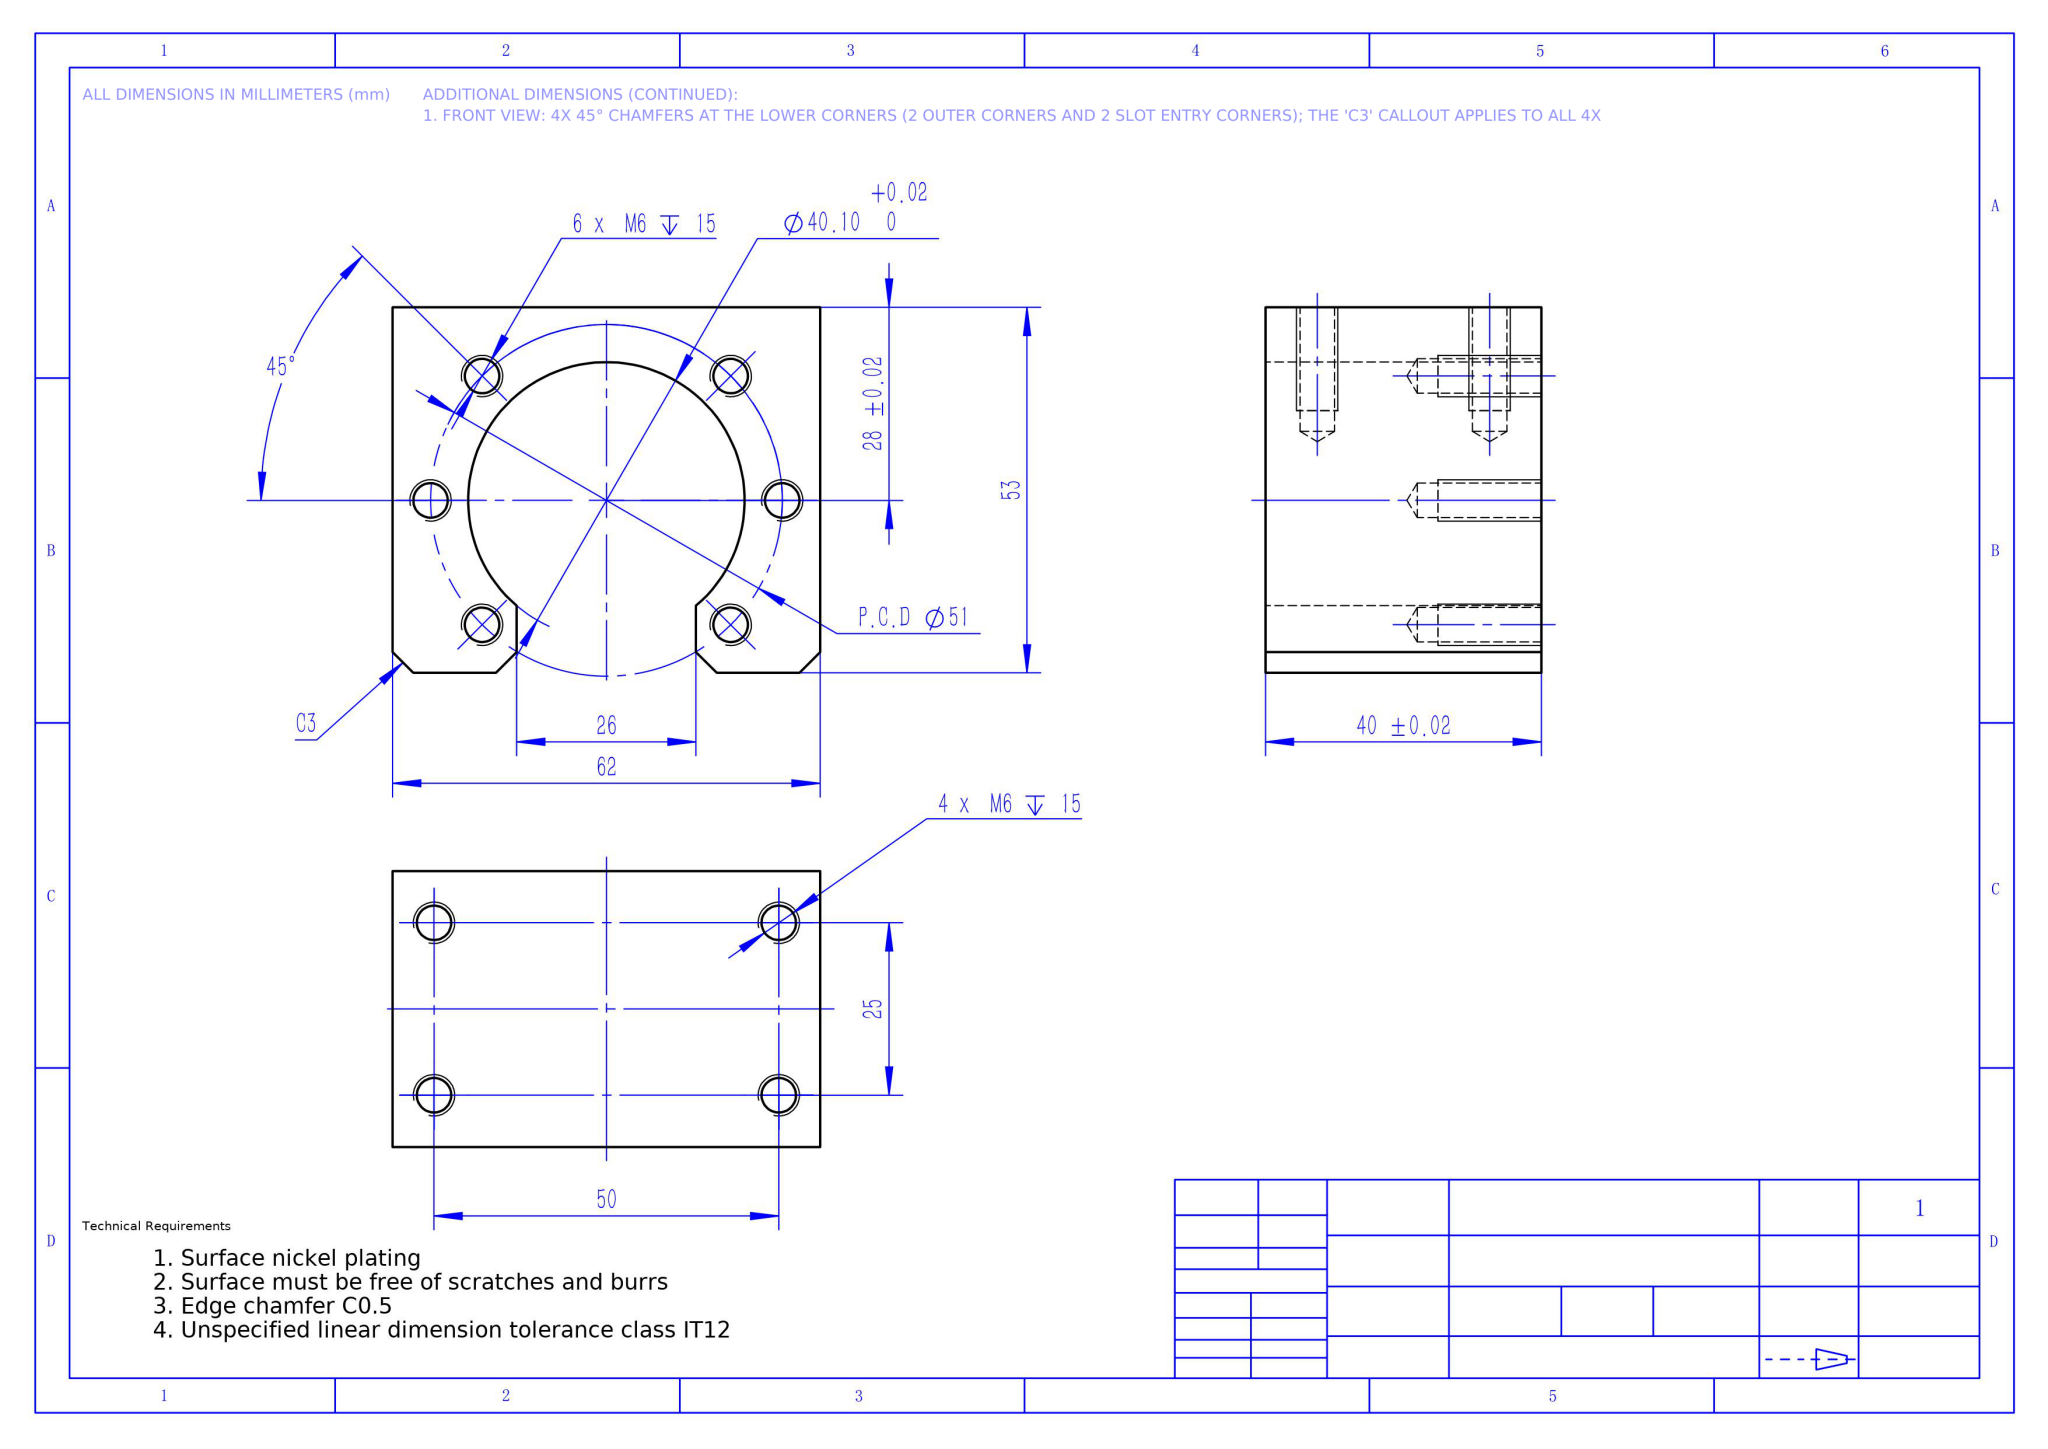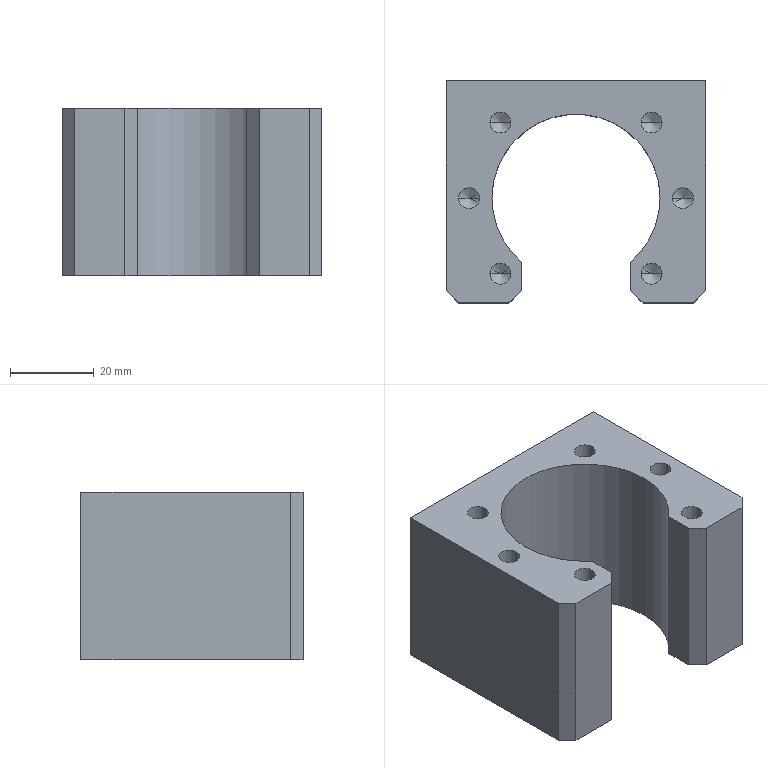Part | NX | mm | 1 solid | 56 faces | box 62 x 53 x 40 mm | volume 69852 mm3 | cylinder 23 | cone 20 | plane 13 | commonest cylinder face diameters 5 x20 40.1 x3